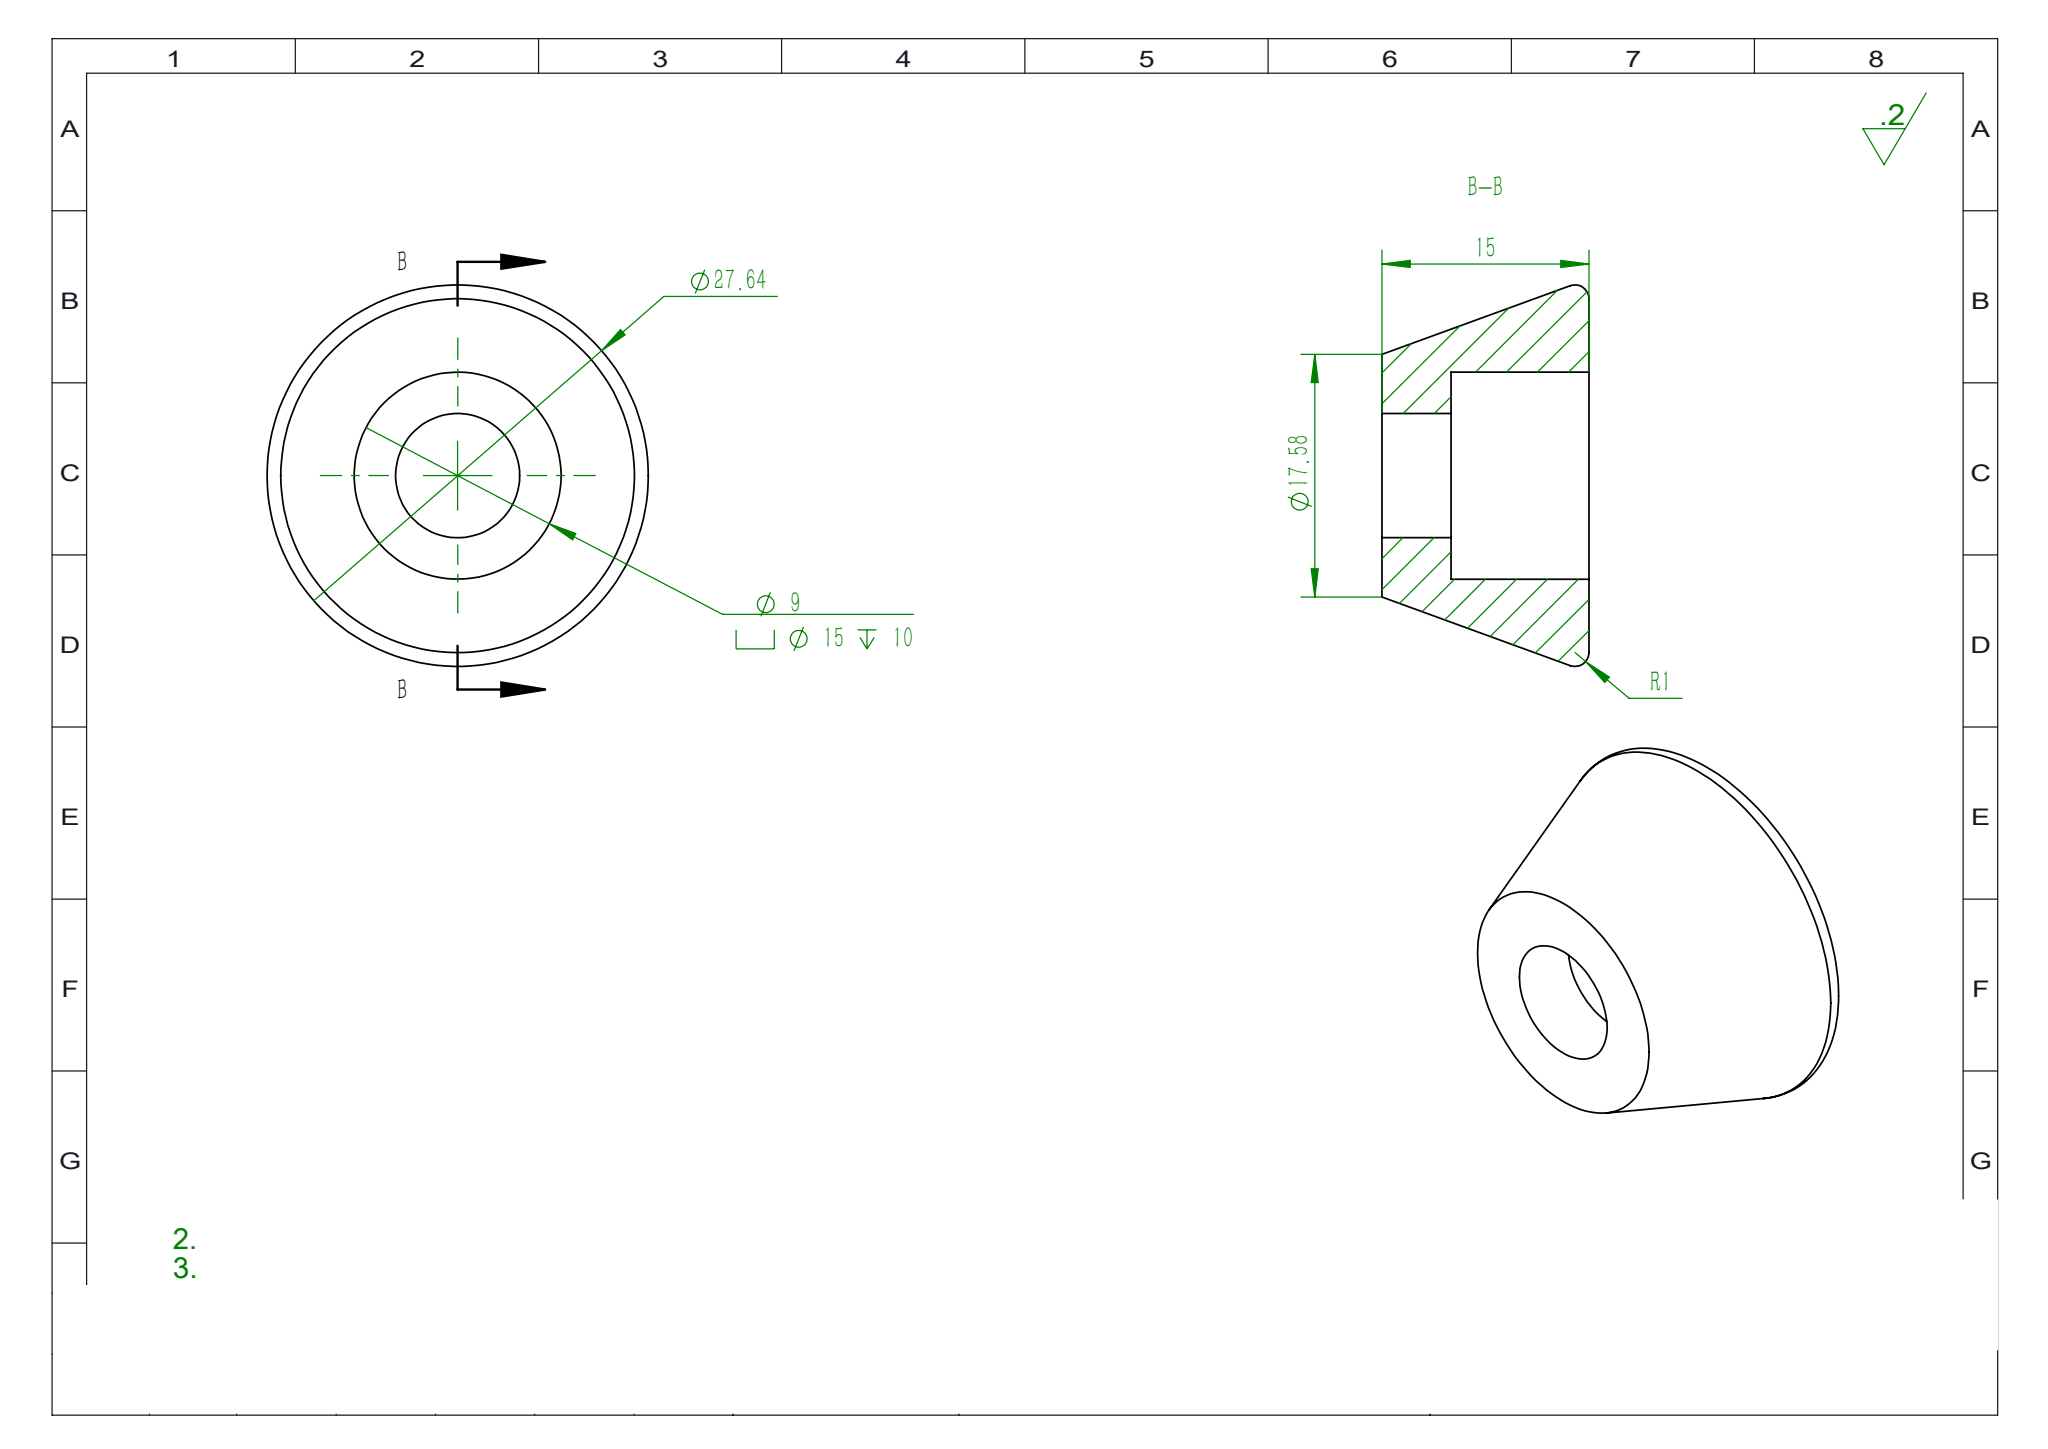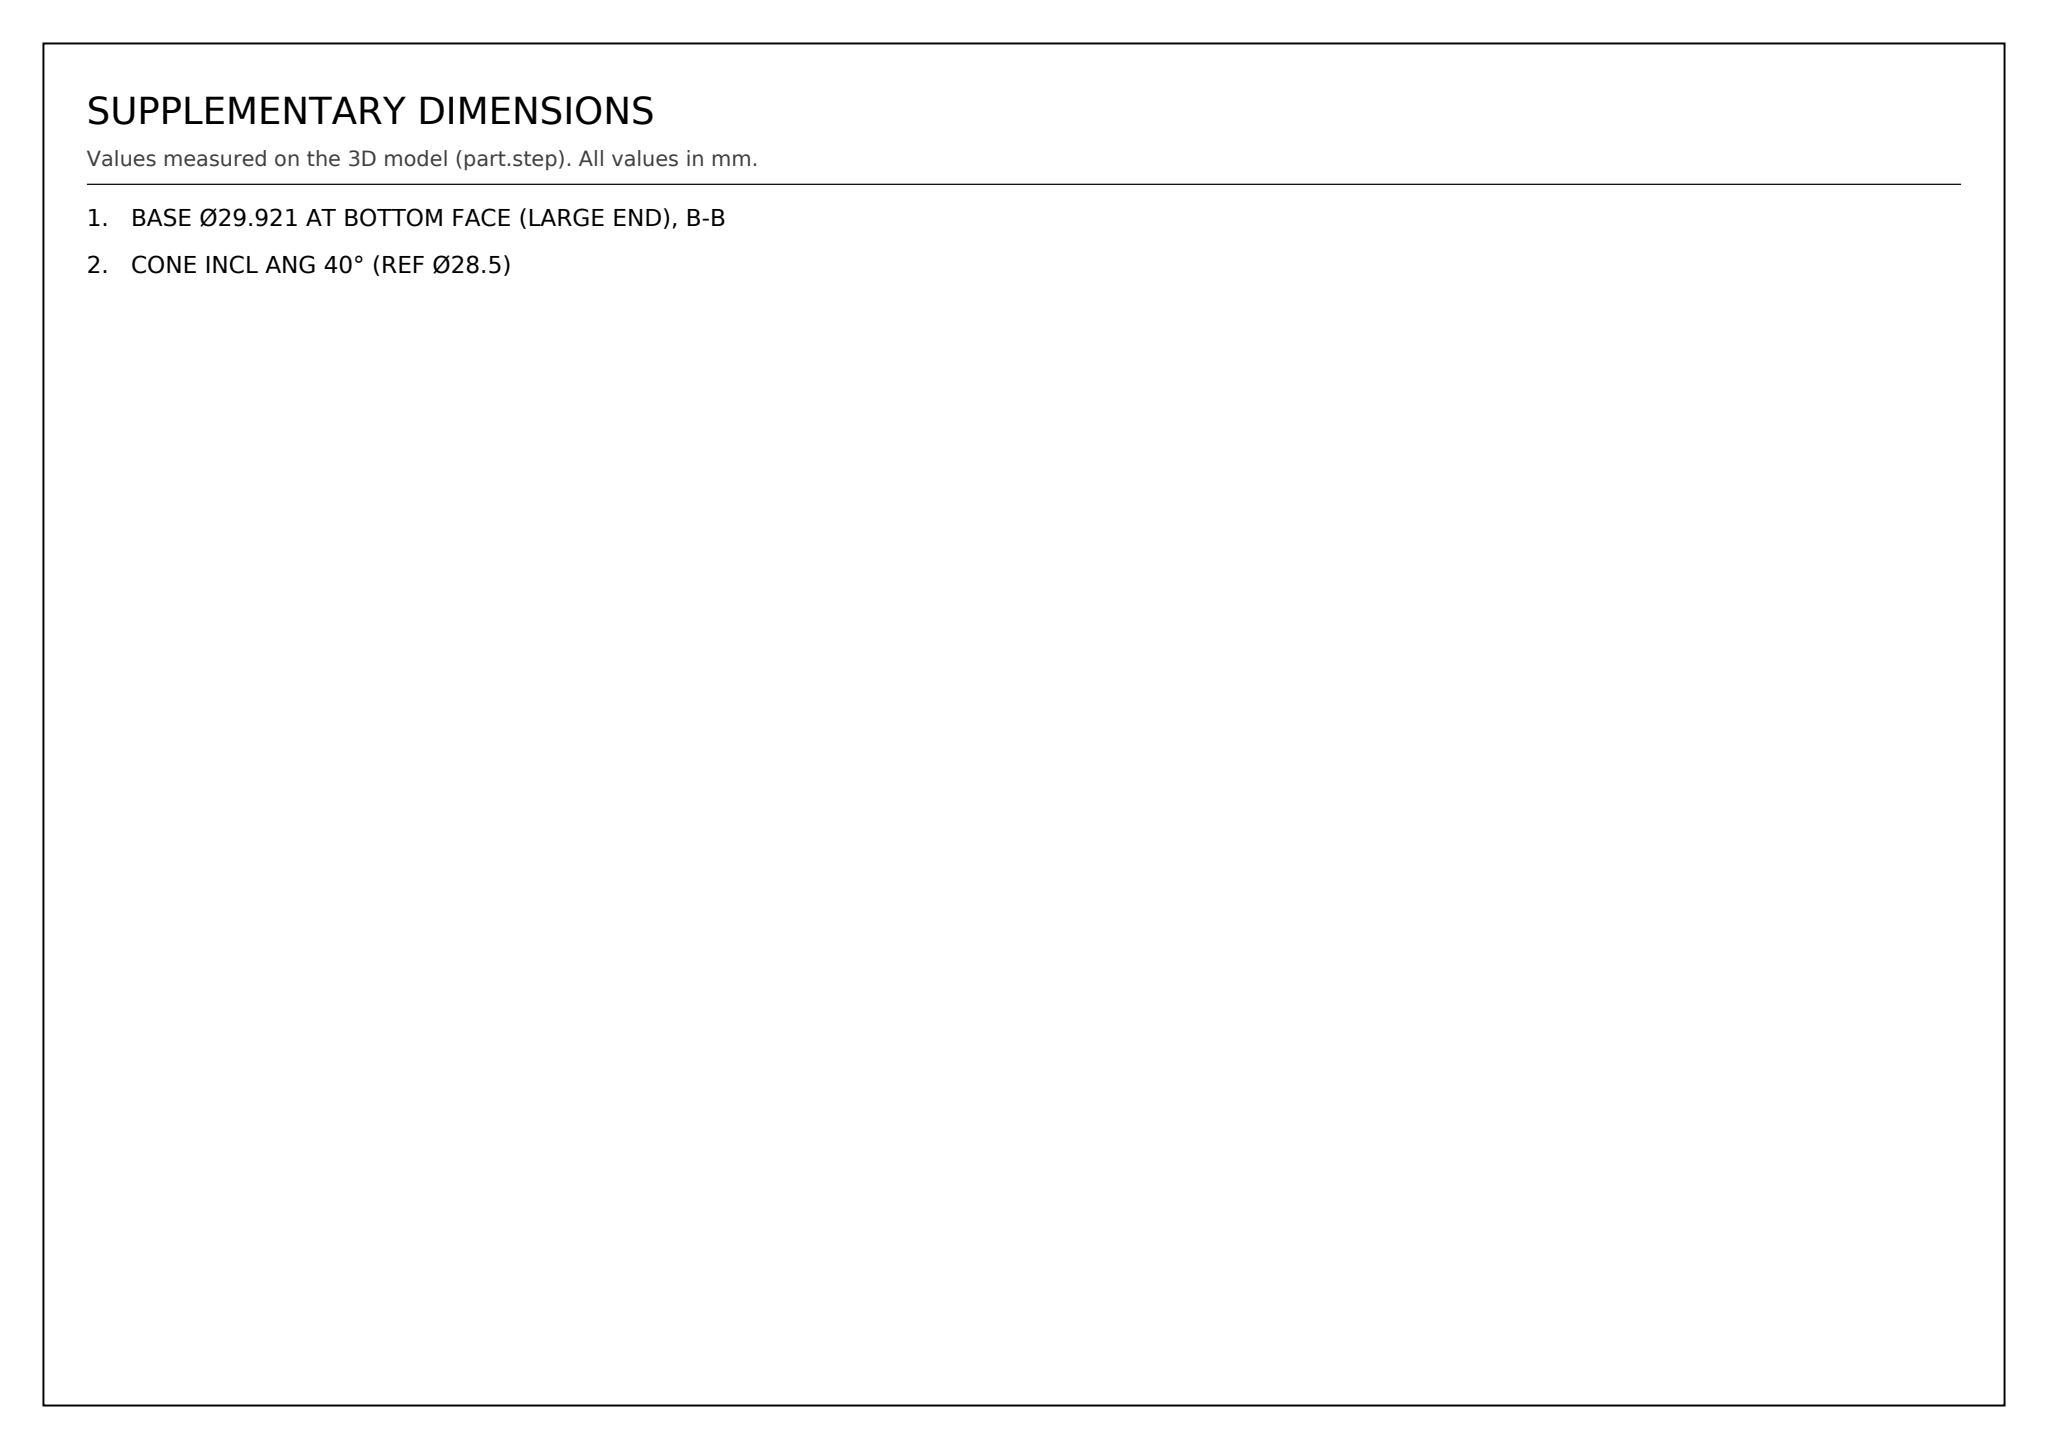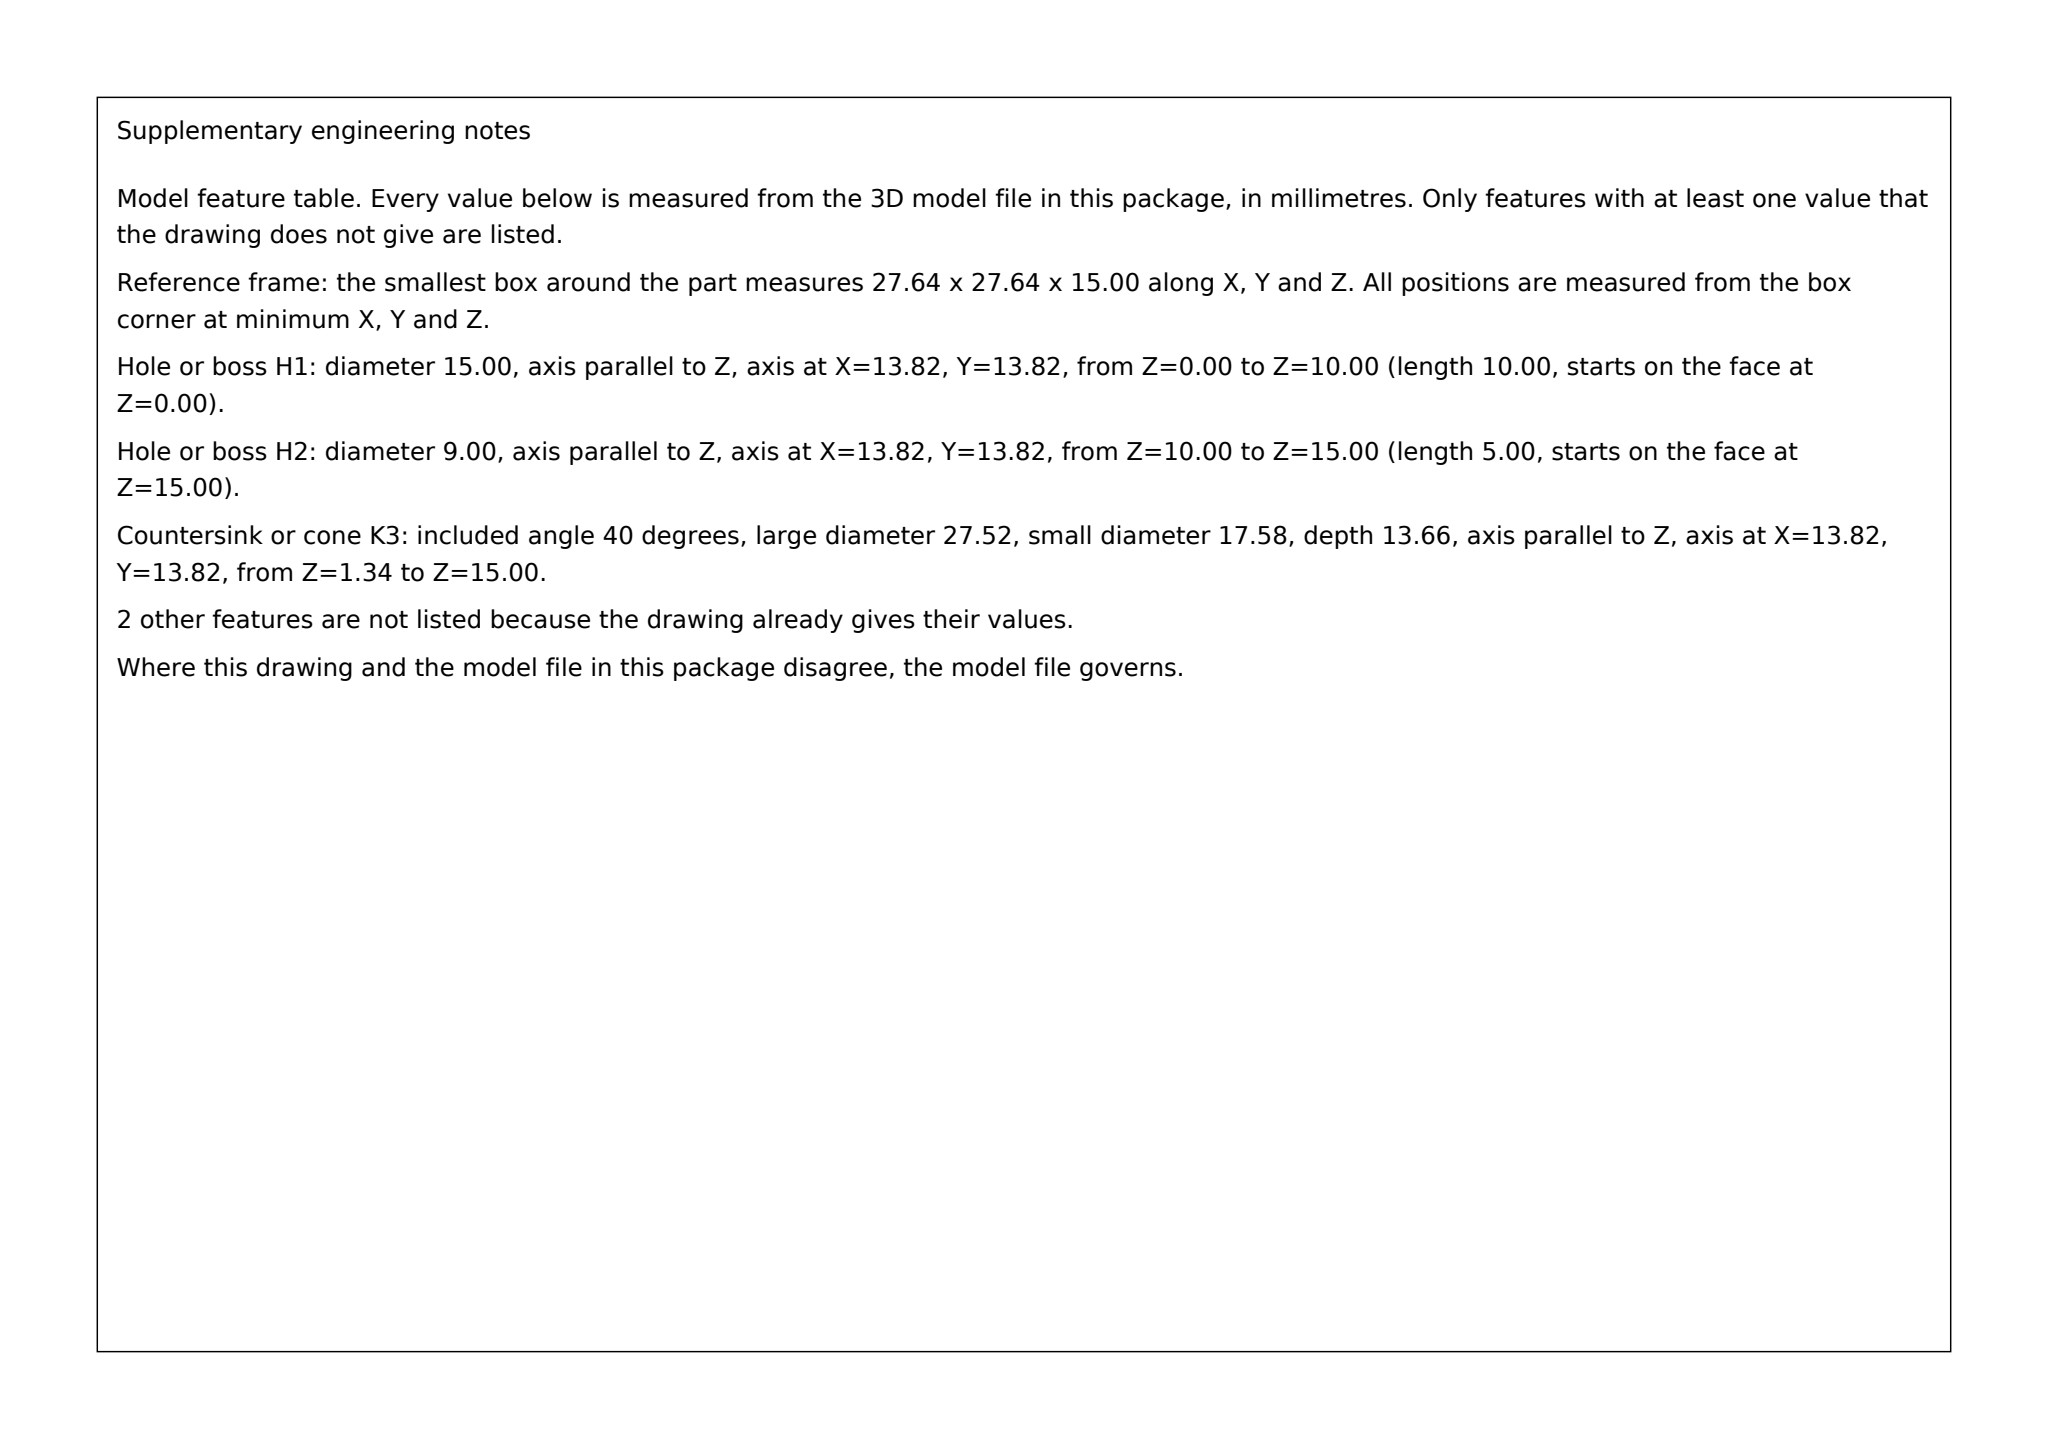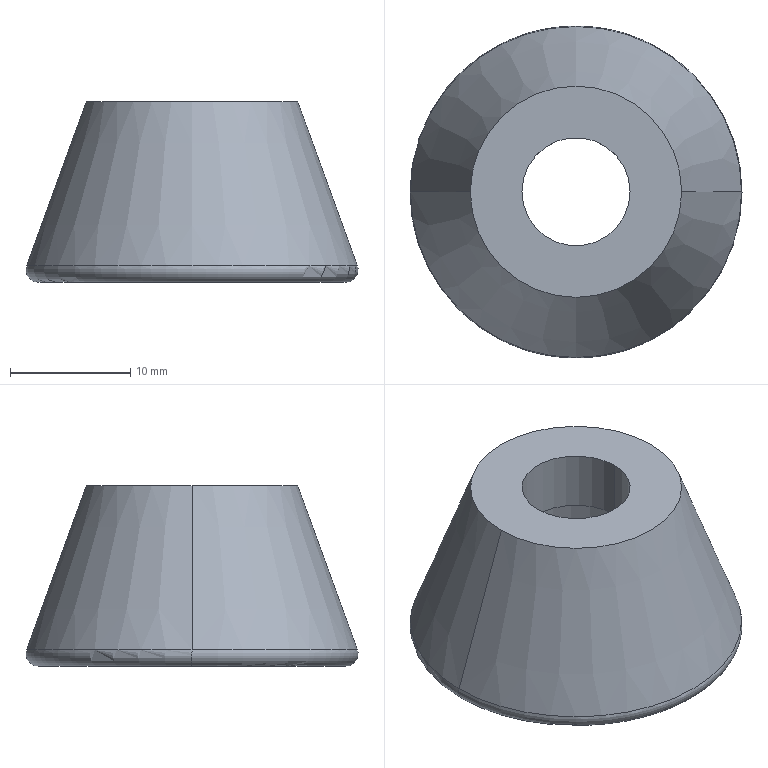Part | SolidWorks | mm | 1 solid | 11 faces | box 27.64 x 27.64 x 15 mm | volume 4245 mm3 | cylinder 4 | plane 3 | torus 2 | cone 2 | commonest cylinder face diameters 15 x2 9 x2
Drawing notes:
BASE Ø29.921 AT BOTTOM FACE (LARGE END), B-B | from the solid: bbox_xyz X/Y = 29.921 max dia at z=0 base face
CONE INCL ANG 40° (REF Ø28.5) | from the solid: cones[included_angle,ref_dia] = [40.0, 28.5]
build123d program:
from build123d import *

# Parameters (mm, degrees)
SKETCH1_R                                       = 14.25
BOSS_EXTRUDE1_DEPTH                             = 15
BOSS_EXTRUDE1_TAPER                             = 20
M8_HEX_SOCKET_HEAD_CAP_SCREW_CBORE1_D           = 9
M8_HEX_SOCKET_HEAD_CAP_SCREW_CBORE1_CBORE_D     = 15
M8_HEX_SOCKET_HEAD_CAP_SCREW_CBORE1_CBORE_DEPTH = 10
FILLET1_R                                       = 1


with BuildPart() as part:
    # Sketch1 → Boss-Extrude1 (new body)
    with BuildSketch(Plane.XY):
        Circle(SKETCH1_R)
    extrude(amount=BOSS_EXTRUDE1_DEPTH, taper=BOSS_EXTRUDE1_TAPER)

    # M8 Hex Socket Head Cap Screw CBORE1 (through all)
    with Locations(Plane(origin=(0, 0, 0), x_dir=(-1, 0, 0), z_dir=(0, 0, -1))):
        with Locations((0, 0)):
            CounterBoreHole(M8_HEX_SOCKET_HEAD_CAP_SCREW_CBORE1_D / 2, M8_HEX_SOCKET_HEAD_CAP_SCREW_CBORE1_CBORE_D / 2, M8_HEX_SOCKET_HEAD_CAP_SCREW_CBORE1_CBORE_DEPTH)

    # Fillet1
    fillet1_edges = [part.edges().sort_by_distance(p)[0] for p in [
        (-14.25, 0, 0),
    ]]
    fillet(fillet1_edges, radius=FILLET1_R)


solid = part.part
STEP:
#1=CARTESIAN_POINT('',(-12.822,0.,0.));
#2=VERTEX_POINT('',#1);
#3=CARTESIAN_POINT('',(12.822,0.,0.));
#4=VERTEX_POINT('',#3);
#5=CARTESIAN_POINT('',(0.,0.,0.));
#6=DIRECTION('',(0.,0.,-1.));
#7=DIRECTION('',(1.,0.,0.));
#8=AXIS2_PLACEMENT_3D('',#5,#6,#7);
#9=CIRCLE('',#8,12.822);
#10=EDGE_CURVE('',#2,#4,#9,.T.);
#11=ORIENTED_EDGE('',*,*,#10,.F.);
#12=CARTESIAN_POINT('',(-13.762,-0.,1.342));
#13=VERTEX_POINT('',#12);
#14=CARTESIAN_POINT('',(-12.822,0.,1.));
#15=DIRECTION('',(0.,1.,0.));
#16=DIRECTION('',(-1.,0.,0.));
#17=AXIS2_PLACEMENT_3D('',#14,#15,#16);
#18=CIRCLE('',#17,1.);
#19=EDGE_CURVE('',#2,#13,#18,.T.);
#20=ORIENTED_EDGE('',*,*,#19,.T.);
#21=CARTESIAN_POINT('',(13.762,0.,1.342));
#22=VERTEX_POINT('',#21);
#23=CARTESIAN_POINT('',(0.,0.,1.342));
#24=DIRECTION('',(0.,0.,1.));
#25=DIRECTION('',(1.,0.,0.));
#26=AXIS2_PLACEMENT_3D('',#23,#24,#25);
#27=CIRCLE('',#26,13.762);
#28=EDGE_CURVE('',#22,#13,#27,.T.);
#29=ORIENTED_EDGE('',*,*,#28,.F.);
#30=CARTESIAN_POINT('',(12.822,0.,1.));
#31=DIRECTION('',(0.,-1.,0.));
#32=DIRECTION('',(0.,0.,-1.));
#33=AXIS2_PLACEMENT_3D('',#30,#31,#32);
#34=CIRCLE('',#33,1.);
#35=EDGE_CURVE('',#4,#22,#34,.T.);
#36=ORIENTED_EDGE('',*,*,#35,.F.);
#37=EDGE_LOOP('',(#11,#20,#29,#36));
#38=FACE_OUTER_BOUND('',#37,.T.);
#39=CARTESIAN_POINT('',(0.,0.,1.));
#40=DIRECTION('',(0.,0.,1.));
#41=DIRECTION('',(1.,0.,0.));
#42=AXIS2_PLACEMENT_3D('',#39,#40,#41);
#43=TOROIDAL_SURFACE('',#42,12.822,1.);
#44=ADVANCED_FACE('',(#38),#43,.T.);
#45=CARTESIAN_POINT('',(7.5,0.,10.));
#46=VERTEX_POINT('',#45);
#47=CARTESIAN_POINT('',(-7.5,0.,10.));
#48=VERTEX_POINT('',#47);
#49=CARTESIAN_POINT('',(0.,0.,10.));
#50=DIRECTION('',(0.,0.,-1.));
#51=DIRECTION('',(-1.,0.,0.));
#52=AXIS2_PLACEMENT_3D('',#49,#50,#51);
#53=CIRCLE('',#52,7.5);
#54=EDGE_CURVE('',#46,#48,#53,.T.);
#55=ORIENTED_EDGE('',*,*,#54,.F.);
#56=CARTESIAN_POINT('',(7.5,0.,0.));
#57=VERTEX_POINT('',#56);
#58=CARTESIAN_POINT('',(7.5,0.,0.));
#59=DIRECTION('',(0.,0.,-1.));
#60=VECTOR('',#59,1000.);
#61=LINE('',#58,#60);
#62=EDGE_CURVE('',#46,#57,#61,.T.);
#63=ORIENTED_EDGE('',*,*,#62,.T.);
#64=CARTESIAN_POINT('',(-7.5,0.,0.));
#65=VERTEX_POINT('',#64);
#66=CARTESIAN_POINT('',(0.,0.,0.));
#67=DIRECTION('',(0.,0.,-1.));
#68=DIRECTION('',(-1.,0.,0.));
#69=AXIS2_PLACEMENT_3D('',#66,#67,#68);
#70=CIRCLE('',#69,7.5);
#71=EDGE_CURVE('',#57,#65,#70,.T.);
#72=ORIENTED_EDGE('',*,*,#71,.T.);
#73=CARTESIAN_POINT('',(-7.5,0.,0.));
#74=DIRECTION('',(0.,0.,-1.));
#75=VECTOR('',#74,1000.);
#76=LINE('',#73,#75);
#77=EDGE_CURVE('',#48,#65,#76,.T.);
#78=ORIENTED_EDGE('',*,*,#77,.F.);
#79=EDGE_LOOP('',(#55,#63,#72,#78));
#80=FACE_OUTER_BOUND('',#79,.T.);
#81=CARTESIAN_POINT('',(0.,0.,0.));
#82=DIRECTION('',(0.,0.,-1.));
#83=DIRECTION('',(-1.,0.,0.));
#84=AXIS2_PLACEMENT_3D('',#81,#82,#83);
#85=CYLINDRICAL_SURFACE('',#84,7.5);
#86=ADVANCED_FACE('',(#80),#85,.F.);
#87=CARTESIAN_POINT('',(4.5,0.,15.));
#88=VERTEX_POINT('',#87);
#89=CARTESIAN_POINT('',(-4.5,0.,15.));
#90=VERTEX_POINT('',#89);
#91=CARTESIAN_POINT('',(0.,0.,15.));
#92=DIRECTION('',(0.,0.,-1.));
#93=DIRECTION('',(-1.,0.,0.));
#94=AXIS2_PLACEMENT_3D('',#91,#92,#93);
#95=CIRCLE('',#94,4.5);
#96=EDGE_CURVE('',#88,#90,#95,.T.);
#97=ORIENTED_EDGE('',*,*,#96,.F.);
#98=CARTESIAN_POINT('',(4.5,0.,10.));
#99=VERTEX_POINT('',#98);
#100=CARTESIAN_POINT('',(4.5,0.,0.));
#101=DIRECTION('',(0.,0.,-1.));
#102=VECTOR('',#101,1000.);
#103=LINE('',#100,#102);
#104=EDGE_CURVE('',#88,#99,#103,.T.);
#105=ORIENTED_EDGE('',*,*,#104,.T.);
#106=CARTESIAN_POINT('',(-4.5,0.,10.));
#107=VERTEX_POINT('',#106);
#108=CARTESIAN_POINT('',(0.,0.,10.));
#109=DIRECTION('',(0.,0.,-1.));
#110=DIRECTION('',(-1.,0.,0.));
#111=AXIS2_PLACEMENT_3D('',#108,#109,#110);
#112=CIRCLE('',#111,4.5);
#113=EDGE_CURVE('',#99,#107,#112,.T.);
#114=ORIENTED_EDGE('',*,*,#113,.T.);
#115=CARTESIAN_POINT('',(-4.5,0.,0.));
#116=DIRECTION('',(0.,0.,-1.));
#117=VECTOR('',#116,1000.);
#118=LINE('',#115,#117);
#119=EDGE_CURVE('',#90,#107,#118,.T.);
#120=ORIENTED_EDGE('',*,*,#119,.F.);
#121=EDGE_LOOP('',(#97,#105,#114,#120));
#122=FACE_OUTER_BOUND('',#121,.T.);
#123=CARTESIAN_POINT('',(0.,0.,0.));
#124=DIRECTION('',(0.,0.,-1.));
#125=DIRECTION('',(-1.,0.,0.));
#126=AXIS2_PLACEMENT_3D('',#123,#124,#125);
#127=CYLINDRICAL_SURFACE('',#126,4.5);
#128=ADVANCED_FACE('',(#122),#127,.F.);
#129=CARTESIAN_POINT('',(-8.79,-0.,15.));
#130=VERTEX_POINT('',#129);
#131=CARTESIAN_POINT('',(8.79,0.,15.));
#132=VERTEX_POINT('',#131);
#133=CARTESIAN_POINT('',(0.,0.,15.));
#134=DIRECTION('',(0.,0.,1.));
#135=DIRECTION('',(1.,0.,0.));
#136=AXIS2_PLACEMENT_3D('',#133,#134,#135);
#137=CIRCLE('',#136,8.79);
#138=EDGE_CURVE('',#130,#132,#137,.T.);
#139=ORIENTED_EDGE('',*,*,#138,.F.);
#140=CARTESIAN_POINT('',(-14.25,-0.,0.));
#141=DIRECTION('',(-0.342,-0.,-0.9397));
#142=VECTOR('',#141,1000.);
#143=LINE('',#140,#142);
#144=EDGE_CURVE('',#130,#13,#143,.T.);
#145=ORIENTED_EDGE('',*,*,#144,.T.);
#146=CARTESIAN_POINT('',(0.,0.,1.342));
#147=DIRECTION('',(0.,0.,1.));
#148=DIRECTION('',(1.,0.,0.));
#149=AXIS2_PLACEMENT_3D('',#146,#147,#148);
#150=CIRCLE('',#149,13.762);
#151=EDGE_CURVE('',#13,#22,#150,.T.);
#152=ORIENTED_EDGE('',*,*,#151,.T.);
#153=CARTESIAN_POINT('',(14.25,0.,0.));
#154=DIRECTION('',(0.342,0.,-0.9397));
#155=VECTOR('',#154,1000.);
#156=LINE('',#153,#155);
#157=EDGE_CURVE('',#132,#22,#156,.T.);
#158=ORIENTED_EDGE('',*,*,#157,.F.);
#159=EDGE_LOOP('',(#139,#145,#152,#158));
#160=FACE_OUTER_BOUND('',#159,.T.);
#161=CARTESIAN_POINT('',(0.,0.,0.));
#162=DIRECTION('',(0.,0.,-1.));
#163=DIRECTION('',(1.,0.,0.));
#164=AXIS2_PLACEMENT_3D('',#161,#162,#163);
#165=CONICAL_SURFACE('',#164,14.25,0.3491);
#166=ADVANCED_FACE('',(#160),#165,.T.);
#167=ORIENTED_EDGE('',*,*,#144,.F.);
#168=CARTESIAN_POINT('',(0.,0.,15.));
#169=DIRECTION('',(0.,0.,1.));
#170=DIRECTION('',(1.,0.,0.));
#171=AXIS2_PLACEMENT_3D('',#168,#169,#170);
#172=CIRCLE('',#171,8.79);
#173=EDGE_CURVE('',#132,#130,#172,.T.);
#174=ORIENTED_EDGE('',*,*,#173,.F.);
#175=ORIENTED_EDGE('',*,*,#157,.T.);
#176=ORIENTED_EDGE('',*,*,#28,.T.);
#177=EDGE_LOOP('',(#167,#174,#175,#176));
#178=FACE_OUTER_BOUND('',#177,.T.);
#179=CARTESIAN_POINT('',(0.,0.,0.));
#180=DIRECTION('',(0.,0.,-1.));
#181=DIRECTION('',(1.,0.,0.));
#182=AXIS2_PLACEMENT_3D('',#179,#180,#181);
#183=CONICAL_SURFACE('',#182,14.25,0.3491);
#184=ADVANCED_FACE('',(#178),#183,.T.);
#185=CARTESIAN_POINT('',(0.,0.,15.));
#186=DIRECTION('',(0.,0.,-1.));
#187=DIRECTION('',(-1.,0.,0.));
#188=AXIS2_PLACEMENT_3D('',#185,#186,#187);
#189=CIRCLE('',#188,4.5);
#190=EDGE_CURVE('',#90,#88,#189,.T.);
#191=ORIENTED_EDGE('',*,*,#190,.T.);
#192=ORIENTED_EDGE('',*,*,#96,.T.);
#193=EDGE_LOOP('',(#191,#192));
#194=FACE_BOUND('',#193,.T.);
#195=ORIENTED_EDGE('',*,*,#173,.T.);
#196=ORIENTED_EDGE('',*,*,#138,.T.);
#197=EDGE_LOOP('',(#195,#196));
#198=FACE_OUTER_BOUND('',#197,.T.);
#199=CARTESIAN_POINT('',(0.,0.,15.));
#200=DIRECTION('',(0.,0.,1.));
#201=DIRECTION('',(1.,0.,0.));
#202=AXIS2_PLACEMENT_3D('',#199,#200,#201);
#203=PLANE('',#202);
#204=ADVANCED_FACE('',(#194,#198),#203,.T.);
#205=CARTESIAN_POINT('',(0.,0.,0.));
#206=DIRECTION('',(0.,0.,-1.));
#207=DIRECTION('',(1.,0.,0.));
#208=AXIS2_PLACEMENT_3D('',#205,#206,#207);
#209=CIRCLE('',#208,12.822);
#210=EDGE_CURVE('',#4,#2,#209,.T.);
#211=ORIENTED_EDGE('',*,*,#210,.T.);
#212=ORIENTED_EDGE('',*,*,#10,.T.);
#213=EDGE_LOOP('',(#211,#212));
#214=FACE_OUTER_BOUND('',#213,.T.);
#215=CARTESIAN_POINT('',(0.,0.,0.));
#216=DIRECTION('',(0.,0.,-1.));
#217=DIRECTION('',(-1.,0.,0.));
#218=AXIS2_PLACEMENT_3D('',#215,#216,#217);
#219=CIRCLE('',#218,7.5);
#220=EDGE_CURVE('',#65,#57,#219,.T.);
#221=ORIENTED_EDGE('',*,*,#220,.F.);
#222=ORIENTED_EDGE('',*,*,#71,.F.);
#223=EDGE_LOOP('',(#221,#222));
#224=FACE_BOUND('',#223,.T.);
#225=CARTESIAN_POINT('',(0.,0.,0.));
#226=DIRECTION('',(0.,0.,1.));
#227=DIRECTION('',(1.,0.,0.));
#228=AXIS2_PLACEMENT_3D('',#225,#226,#227);
#229=PLANE('',#228);
#230=ADVANCED_FACE('',(#214,#224),#229,.F.);
#231=ORIENTED_EDGE('',*,*,#104,.F.);
#232=ORIENTED_EDGE('',*,*,#190,.F.);
#233=ORIENTED_EDGE('',*,*,#119,.T.);
#234=CARTESIAN_POINT('',(0.,0.,10.));
#235=DIRECTION('',(0.,0.,-1.));
#236=DIRECTION('',(-1.,0.,0.));
#237=AXIS2_PLACEMENT_3D('',#234,#235,#236);
#238=CIRCLE('',#237,4.5);
#239=EDGE_CURVE('',#107,#99,#238,.T.);
#240=ORIENTED_EDGE('',*,*,#239,.T.);
#241=EDGE_LOOP('',(#231,#232,#233,#240));
#242=FACE_OUTER_BOUND('',#241,.T.);
#243=CARTESIAN_POINT('',(0.,0.,0.));
#244=DIRECTION('',(0.,0.,-1.));
#245=DIRECTION('',(-1.,0.,0.));
#246=AXIS2_PLACEMENT_3D('',#243,#244,#245);
#247=CYLINDRICAL_SURFACE('',#246,4.5);
#248=ADVANCED_FACE('',(#242),#247,.F.);
#249=ORIENTED_EDGE('',*,*,#239,.F.);
#250=ORIENTED_EDGE('',*,*,#113,.F.);
#251=EDGE_LOOP('',(#249,#250));
#252=FACE_BOUND('',#251,.T.);
#253=CARTESIAN_POINT('',(0.,0.,10.));
#254=DIRECTION('',(0.,0.,-1.));
#255=DIRECTION('',(-1.,0.,0.));
#256=AXIS2_PLACEMENT_3D('',#253,#254,#255);
#257=CIRCLE('',#256,7.5);
#258=EDGE_CURVE('',#48,#46,#257,.T.);
#259=ORIENTED_EDGE('',*,*,#258,.T.);
#260=ORIENTED_EDGE('',*,*,#54,.T.);
#261=EDGE_LOOP('',(#259,#260));
#262=FACE_OUTER_BOUND('',#261,.T.);
#263=CARTESIAN_POINT('',(4.5,0.,10.));
#264=DIRECTION('',(0.,0.,1.));
#265=DIRECTION('',(1.,0.,0.));
#266=AXIS2_PLACEMENT_3D('',#263,#264,#265);
#267=PLANE('',#266);
#268=ADVANCED_FACE('',(#252,#262),#267,.F.);
#269=ORIENTED_EDGE('',*,*,#62,.F.);
#270=ORIENTED_EDGE('',*,*,#258,.F.);
#271=ORIENTED_EDGE('',*,*,#77,.T.);
#272=ORIENTED_EDGE('',*,*,#220,.T.);
#273=EDGE_LOOP('',(#269,#270,#271,#272));
#274=FACE_OUTER_BOUND('',#273,.T.);
#275=CARTESIAN_POINT('',(0.,0.,0.));
#276=DIRECTION('',(0.,0.,-1.));
#277=DIRECTION('',(-1.,0.,0.));
#278=AXIS2_PLACEMENT_3D('',#275,#276,#277);
#279=CYLINDRICAL_SURFACE('',#278,7.5);
#280=ADVANCED_FACE('',(#274),#279,.F.);
#281=ORIENTED_EDGE('',*,*,#19,.F.);
#282=ORIENTED_EDGE('',*,*,#210,.F.);
#283=ORIENTED_EDGE('',*,*,#35,.T.);
#284=ORIENTED_EDGE('',*,*,#151,.F.);
#285=EDGE_LOOP('',(#281,#282,#283,#284));
#286=FACE_OUTER_BOUND('',#285,.T.);
#287=CARTESIAN_POINT('',(0.,0.,1.));
#288=DIRECTION('',(0.,0.,1.));
#289=DIRECTION('',(1.,0.,0.));
#290=AXIS2_PLACEMENT_3D('',#287,#288,#289);
#291=TOROIDAL_SURFACE('',#290,12.822,1.);
#292=ADVANCED_FACE('',(#286),#291,.T.);
#293=CLOSED_SHELL('',(#44,#86,#128,#166,#184,#204,#230,#248,#268,#280,#292));
#294=MANIFOLD_SOLID_BREP('',#293);
#295=CARTESIAN_POINT('',(0.,0.,0.));
#296=DIRECTION('',(0.,0.,1.));
#297=DIRECTION('',(1.,0.,0.));
#298=AXIS2_PLACEMENT_3D('',#295,#296,#297);
#299=(LENGTH_UNIT()NAMED_UNIT(*)SI_UNIT(.MILLI.,.METRE.));
#300=UNCERTAINTY_MEASURE_WITH_UNIT(LENGTH_MEASURE(0.00001),#299,'','');
#301=(NAMED_UNIT(*)PLANE_ANGLE_UNIT()SI_UNIT($,.RADIAN.));
#302=(NAMED_UNIT(*)SI_UNIT($,.STERADIAN.)SOLID_ANGLE_UNIT());
#303=(GEOMETRIC_REPRESENTATION_CONTEXT(3)GLOBAL_UNCERTAINTY_ASSIGNED_CONTEXT((#300))GLOBAL_UNIT_ASSIGNED_CONTEXT((#299,#301,#302))REPRESENTATION_CONTEXT('',''));
#304=ADVANCED_BREP_SHAPE_REPRESENTATION('',(#294,#298),#303);